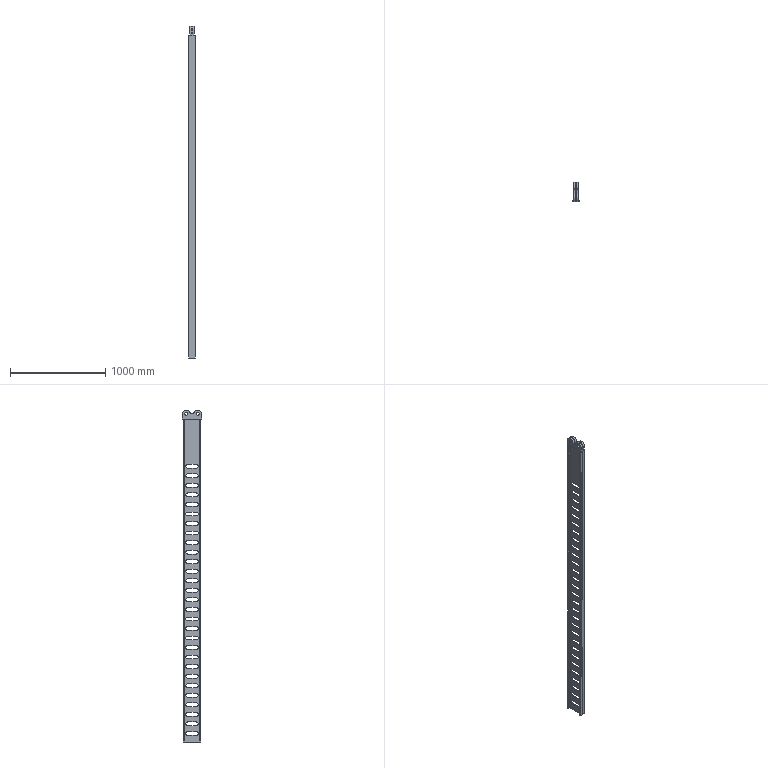Component | NX | MID_BEAM | 1 solid | 158 faces | volume 6156541 mm3 | plane 92 | cylinder 66 | commonest cylinder face diameters 40 x58 80 x4 30 x4